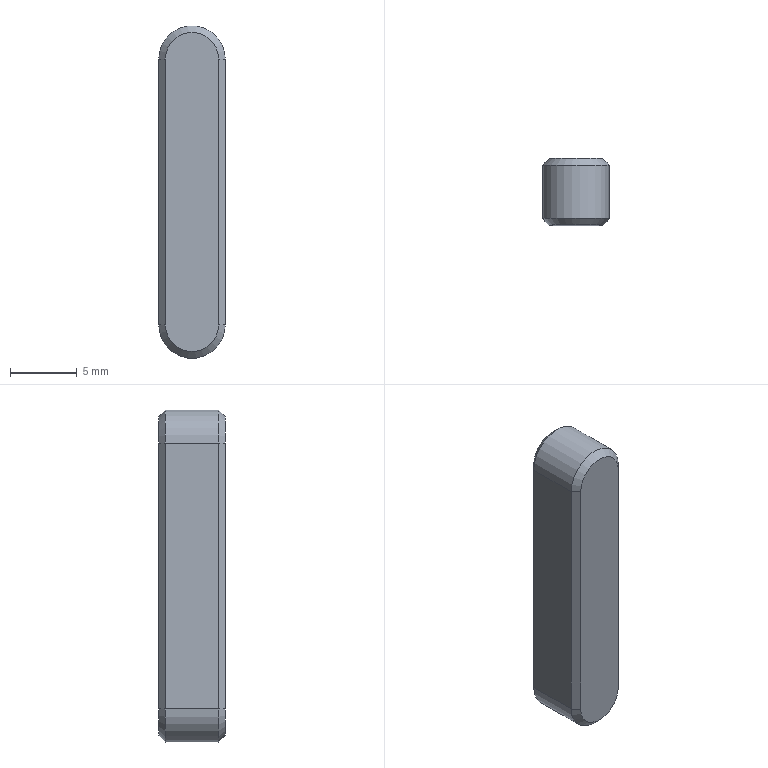Component | SolidWorks | 25x5x5ParallelKey-1 | 1 solid | 14 faces | box 5 x 5 x 25 mm | volume 585 mm3 | plane 8 | cone 4 | cylinder 2 | commonest cylinder face diameters 5 x2 | material AISI 1045 Steel, cold drawn
build123d program:
from build123d import *

# Parameters (mm, degrees)
BOSS_EXTRUDE1_DEPTH = 2.5
CHAMFER1_SIZE       = 0.5


with BuildPart() as part:
    # Sketch1 → Boss-Extrude1 (new, symmetric)
    with BuildSketch(Plane.XY):
        with BuildLine():
            Line((-2.5, -10), (-2.5, 10))
            ThreePointArc((-2.5, 10), (0, 12.5), (2.5, 10))
            Line((2.5, 10), (2.5, -10))
            ThreePointArc((2.5, -10), (0, -12.5), (-2.5, -10))
        make_face()
    extrude(amount=BOSS_EXTRUDE1_DEPTH, both=True)

    # Chamfer1
    chamfer1_edges = [part.edges().sort_by_distance(p)[0] for p in [
        (0, 12.5, 2.5),
        (-2.5, 0, 2.5),
        (0, -12.5, 2.5),
        (-2.5, 0, -2.5),
        (0, 12.5, -2.5),
        (2.5, 0, -2.5),
        (0, -12.5, -2.5),
        (2.5, 0, 2.5),
    ]]
    chamfer(chamfer1_edges, length=CHAMFER1_SIZE)


solid = part.part

# Placed as in the assembly
solid = solid.moved(Location((0, 7.5, 115.5), (90, 0, 0)))
STEP:
#1=CARTESIAN_POINT('',(-0.09843,0.2165,4.154));
#2=VERTEX_POINT('',#1);
#3=CARTESIAN_POINT('',(-0.09843,0.374,4.154));
#4=VERTEX_POINT('',#3);
#5=CARTESIAN_POINT('',(-0.09843,0.1969,4.154));
#6=DIRECTION('',(-0.,1.,-0.));
#7=VECTOR('',#6,39.37);
#8=LINE('',#5,#7);
#9=EDGE_CURVE('',#2,#4,#8,.T.);
#10=ORIENTED_EDGE('',*,*,#9,.T.);
#11=CARTESIAN_POINT('',(0.09843,0.374,4.154));
#12=VERTEX_POINT('',#11);
#13=CARTESIAN_POINT('',(-0.,0.374,4.154));
#14=DIRECTION('',(0.,-1.,0.));
#15=DIRECTION('',(1.,0.,0.));
#16=AXIS2_PLACEMENT_3D('',#13,#14,#15);
#17=CIRCLE('',#16,0.09843);
#18=EDGE_CURVE('',#4,#12,#17,.T.);
#19=ORIENTED_EDGE('',*,*,#18,.T.);
#20=CARTESIAN_POINT('',(0.09843,0.2165,4.154));
#21=VERTEX_POINT('',#20);
#22=CARTESIAN_POINT('',(0.09843,0.1969,4.154));
#23=DIRECTION('',(-0.,1.,-0.));
#24=VECTOR('',#23,39.37);
#25=LINE('',#22,#24);
#26=EDGE_CURVE('',#21,#12,#25,.T.);
#27=ORIENTED_EDGE('',*,*,#26,.F.);
#28=CARTESIAN_POINT('',(0.,0.2165,4.154));
#29=DIRECTION('',(-0.,1.,-0.));
#30=DIRECTION('',(1.,0.,0.));
#31=AXIS2_PLACEMENT_3D('',#28,#29,#30);
#32=CIRCLE('',#31,0.09843);
#33=EDGE_CURVE('',#21,#2,#32,.T.);
#34=ORIENTED_EDGE('',*,*,#33,.T.);
#35=EDGE_LOOP('',(#10,#19,#27,#34));
#36=FACE_OUTER_BOUND('',#35,.T.);
#37=CARTESIAN_POINT('',(0.,0.1969,4.154));
#38=DIRECTION('',(-0.,1.,-0.));
#39=DIRECTION('',(-1.,-0.,0.));
#40=AXIS2_PLACEMENT_3D('',#37,#38,#39);
#41=CYLINDRICAL_SURFACE('',#40,0.09843);
#42=ADVANCED_FACE('',(#36),#41,.T.);
#43=ORIENTED_EDGE('',*,*,#26,.T.);
#44=CARTESIAN_POINT('',(0.09843,0.374,4.941));
#45=VERTEX_POINT('',#44);
#46=CARTESIAN_POINT('',(0.09843,0.374,4.154));
#47=DIRECTION('',(0.,0.,1.));
#48=VECTOR('',#47,39.37);
#49=LINE('',#46,#48);
#50=EDGE_CURVE('',#12,#45,#49,.T.);
#51=ORIENTED_EDGE('',*,*,#50,.T.);
#52=CARTESIAN_POINT('',(0.09843,0.2165,4.941));
#53=VERTEX_POINT('',#52);
#54=CARTESIAN_POINT('',(0.09843,0.1969,4.941));
#55=DIRECTION('',(-0.,1.,-0.));
#56=VECTOR('',#55,39.37);
#57=LINE('',#54,#56);
#58=EDGE_CURVE('',#53,#45,#57,.T.);
#59=ORIENTED_EDGE('',*,*,#58,.F.);
#60=CARTESIAN_POINT('',(0.09843,0.2165,4.154));
#61=DIRECTION('',(-0.,-0.,-1.));
#62=VECTOR('',#61,39.37);
#63=LINE('',#60,#62);
#64=EDGE_CURVE('',#53,#21,#63,.T.);
#65=ORIENTED_EDGE('',*,*,#64,.T.);
#66=EDGE_LOOP('',(#43,#51,#59,#65));
#67=FACE_OUTER_BOUND('',#66,.T.);
#68=CARTESIAN_POINT('',(0.09843,0.1969,4.154));
#69=DIRECTION('',(-1.,-0.,0.));
#70=DIRECTION('',(-0.,-0.,-1.));
#71=AXIS2_PLACEMENT_3D('',#68,#69,#70);
#72=PLANE('',#71);
#73=ADVANCED_FACE('',(#67),#72,.F.);
#74=ORIENTED_EDGE('',*,*,#58,.T.);
#75=CARTESIAN_POINT('',(-0.09843,0.374,4.941));
#76=VERTEX_POINT('',#75);
#77=CARTESIAN_POINT('',(-0.,0.374,4.941));
#78=DIRECTION('',(0.,-1.,0.));
#79=DIRECTION('',(1.,0.,0.));
#80=AXIS2_PLACEMENT_3D('',#77,#78,#79);
#81=CIRCLE('',#80,0.09843);
#82=EDGE_CURVE('',#45,#76,#81,.T.);
#83=ORIENTED_EDGE('',*,*,#82,.T.);
#84=CARTESIAN_POINT('',(-0.09843,0.2165,4.941));
#85=VERTEX_POINT('',#84);
#86=CARTESIAN_POINT('',(-0.09843,0.1969,4.941));
#87=DIRECTION('',(-0.,1.,-0.));
#88=VECTOR('',#87,39.37);
#89=LINE('',#86,#88);
#90=EDGE_CURVE('',#85,#76,#89,.T.);
#91=ORIENTED_EDGE('',*,*,#90,.F.);
#92=CARTESIAN_POINT('',(0.,0.2165,4.941));
#93=DIRECTION('',(-0.,1.,-0.));
#94=DIRECTION('',(1.,0.,0.));
#95=AXIS2_PLACEMENT_3D('',#92,#93,#94);
#96=CIRCLE('',#95,0.09843);
#97=EDGE_CURVE('',#85,#53,#96,.T.);
#98=ORIENTED_EDGE('',*,*,#97,.T.);
#99=EDGE_LOOP('',(#74,#83,#91,#98));
#100=FACE_OUTER_BOUND('',#99,.T.);
#101=CARTESIAN_POINT('',(0.,0.1969,4.941));
#102=DIRECTION('',(-0.,1.,-0.));
#103=DIRECTION('',(-1.,-0.,0.));
#104=AXIS2_PLACEMENT_3D('',#101,#102,#103);
#105=CYLINDRICAL_SURFACE('',#104,0.09843);
#106=ADVANCED_FACE('',(#100),#105,.T.);
#107=ORIENTED_EDGE('',*,*,#90,.T.);
#108=CARTESIAN_POINT('',(-0.09843,0.374,4.154));
#109=DIRECTION('',(-0.,-0.,-1.));
#110=VECTOR('',#109,39.37);
#111=LINE('',#108,#110);
#112=EDGE_CURVE('',#76,#4,#111,.T.);
#113=ORIENTED_EDGE('',*,*,#112,.T.);
#114=ORIENTED_EDGE('',*,*,#9,.F.);
#115=CARTESIAN_POINT('',(-0.09843,0.2165,4.941));
#116=DIRECTION('',(0.,0.,1.));
#117=VECTOR('',#116,39.37);
#118=LINE('',#115,#117);
#119=EDGE_CURVE('',#2,#85,#118,.T.);
#120=ORIENTED_EDGE('',*,*,#119,.T.);
#121=EDGE_LOOP('',(#107,#113,#114,#120));
#122=FACE_OUTER_BOUND('',#121,.T.);
#123=CARTESIAN_POINT('',(-0.09843,0.1969,4.154));
#124=DIRECTION('',(1.,0.,-0.));
#125=DIRECTION('',(0.,0.,1.));
#126=AXIS2_PLACEMENT_3D('',#123,#124,#125);
#127=PLANE('',#126);
#128=ADVANCED_FACE('',(#122),#127,.F.);
#129=CARTESIAN_POINT('',(0.07874,0.1969,4.941));
#130=VERTEX_POINT('',#129);
#131=CARTESIAN_POINT('',(-0.07874,0.1969,4.941));
#132=VERTEX_POINT('',#131);
#133=CARTESIAN_POINT('',(0.,0.1969,4.941));
#134=DIRECTION('',(0.,-1.,0.));
#135=DIRECTION('',(1.,0.,0.));
#136=AXIS2_PLACEMENT_3D('',#133,#134,#135);
#137=CIRCLE('',#136,0.07874);
#138=EDGE_CURVE('',#130,#132,#137,.T.);
#139=ORIENTED_EDGE('',*,*,#138,.T.);
#140=CARTESIAN_POINT('',(-0.07874,0.1969,4.154));
#141=VERTEX_POINT('',#140);
#142=CARTESIAN_POINT('',(-0.07874,0.1969,4.154));
#143=DIRECTION('',(-0.,-0.,-1.));
#144=VECTOR('',#143,39.37);
#145=LINE('',#142,#144);
#146=EDGE_CURVE('',#132,#141,#145,.T.);
#147=ORIENTED_EDGE('',*,*,#146,.T.);
#148=CARTESIAN_POINT('',(0.07874,0.1969,4.154));
#149=VERTEX_POINT('',#148);
#150=CARTESIAN_POINT('',(0.,0.1969,4.154));
#151=DIRECTION('',(0.,-1.,0.));
#152=DIRECTION('',(1.,0.,0.));
#153=AXIS2_PLACEMENT_3D('',#150,#151,#152);
#154=CIRCLE('',#153,0.07874);
#155=EDGE_CURVE('',#141,#149,#154,.T.);
#156=ORIENTED_EDGE('',*,*,#155,.T.);
#157=CARTESIAN_POINT('',(0.07874,0.1969,4.941));
#158=DIRECTION('',(0.,0.,1.));
#159=VECTOR('',#158,39.37);
#160=LINE('',#157,#159);
#161=EDGE_CURVE('',#149,#130,#160,.T.);
#162=ORIENTED_EDGE('',*,*,#161,.T.);
#163=EDGE_LOOP('',(#139,#147,#156,#162));
#164=FACE_OUTER_BOUND('',#163,.T.);
#165=CARTESIAN_POINT('',(0.,0.1969,4.154));
#166=DIRECTION('',(0.,-1.,0.));
#167=DIRECTION('',(1.,0.,-0.));
#168=AXIS2_PLACEMENT_3D('',#165,#166,#167);
#169=PLANE('',#168);
#170=ADVANCED_FACE('',(#164),#169,.T.);
#171=CARTESIAN_POINT('',(-0.07874,0.3937,4.941));
#172=VERTEX_POINT('',#171);
#173=CARTESIAN_POINT('',(0.07874,0.3937,4.941));
#174=VERTEX_POINT('',#173);
#175=CARTESIAN_POINT('',(-0.,0.3937,4.941));
#176=DIRECTION('',(-0.,1.,-0.));
#177=DIRECTION('',(1.,0.,0.));
#178=AXIS2_PLACEMENT_3D('',#175,#176,#177);
#179=CIRCLE('',#178,0.07874);
#180=EDGE_CURVE('',#172,#174,#179,.T.);
#181=ORIENTED_EDGE('',*,*,#180,.T.);
#182=CARTESIAN_POINT('',(0.07874,0.3937,4.154));
#183=VERTEX_POINT('',#182);
#184=CARTESIAN_POINT('',(0.07874,0.3937,4.154));
#185=DIRECTION('',(-0.,-0.,-1.));
#186=VECTOR('',#185,39.37);
#187=LINE('',#184,#186);
#188=EDGE_CURVE('',#174,#183,#187,.T.);
#189=ORIENTED_EDGE('',*,*,#188,.T.);
#190=CARTESIAN_POINT('',(-0.07874,0.3937,4.154));
#191=VERTEX_POINT('',#190);
#192=CARTESIAN_POINT('',(-0.,0.3937,4.154));
#193=DIRECTION('',(-0.,1.,-0.));
#194=DIRECTION('',(1.,0.,0.));
#195=AXIS2_PLACEMENT_3D('',#192,#193,#194);
#196=CIRCLE('',#195,0.07874);
#197=EDGE_CURVE('',#183,#191,#196,.T.);
#198=ORIENTED_EDGE('',*,*,#197,.T.);
#199=CARTESIAN_POINT('',(-0.07874,0.3937,4.154));
#200=DIRECTION('',(0.,0.,1.));
#201=VECTOR('',#200,39.37);
#202=LINE('',#199,#201);
#203=EDGE_CURVE('',#191,#172,#202,.T.);
#204=ORIENTED_EDGE('',*,*,#203,.T.);
#205=EDGE_LOOP('',(#181,#189,#198,#204));
#206=FACE_OUTER_BOUND('',#205,.T.);
#207=CARTESIAN_POINT('',(-0.,0.3937,4.154));
#208=DIRECTION('',(0.,-1.,0.));
#209=DIRECTION('',(1.,0.,-0.));
#210=AXIS2_PLACEMENT_3D('',#207,#208,#209);
#211=PLANE('',#210);
#212=ADVANCED_FACE('',(#206),#211,.F.);
#213=CARTESIAN_POINT('',(-0.07874,0.3937,4.941));
#214=DIRECTION('',(-0.7071,-0.7071,0.));
#215=VECTOR('',#214,39.37);
#216=LINE('',#213,#215);
#217=EDGE_CURVE('',#172,#76,#216,.T.);
#218=ORIENTED_EDGE('',*,*,#217,.F.);
#219=ORIENTED_EDGE('',*,*,#203,.F.);
#220=CARTESIAN_POINT('',(-0.09843,0.374,4.154));
#221=DIRECTION('',(0.7071,0.7071,-0.));
#222=VECTOR('',#221,39.37);
#223=LINE('',#220,#222);
#224=EDGE_CURVE('',#4,#191,#223,.T.);
#225=ORIENTED_EDGE('',*,*,#224,.F.);
#226=ORIENTED_EDGE('',*,*,#112,.F.);
#227=EDGE_LOOP('',(#218,#219,#225,#226));
#228=FACE_OUTER_BOUND('',#227,.T.);
#229=CARTESIAN_POINT('',(-0.09843,0.374,4.154));
#230=DIRECTION('',(0.7071,-0.7071,-0.));
#231=DIRECTION('',(-0.,-0.,-1.));
#232=AXIS2_PLACEMENT_3D('',#229,#230,#231);
#233=PLANE('',#232);
#234=ADVANCED_FACE('',(#228),#233,.F.);
#235=ORIENTED_EDGE('',*,*,#224,.T.);
#236=ORIENTED_EDGE('',*,*,#197,.F.);
#237=CARTESIAN_POINT('',(0.09843,0.374,4.154));
#238=DIRECTION('',(-0.7071,0.7071,0.));
#239=VECTOR('',#238,39.37);
#240=LINE('',#237,#239);
#241=EDGE_CURVE('',#12,#183,#240,.T.);
#242=ORIENTED_EDGE('',*,*,#241,.F.);
#243=ORIENTED_EDGE('',*,*,#18,.F.);
#244=EDGE_LOOP('',(#235,#236,#242,#243));
#245=FACE_OUTER_BOUND('',#244,.T.);
#246=CARTESIAN_POINT('',(-0.,0.374,4.154));
#247=DIRECTION('',(0.,-1.,0.));
#248=DIRECTION('',(1.,0.,0.));
#249=AXIS2_PLACEMENT_3D('',#246,#247,#248);
#250=CONICAL_SURFACE('',#249,0.09843,0.7854);
#251=ADVANCED_FACE('',(#245),#250,.T.);
#252=ORIENTED_EDGE('',*,*,#217,.T.);
#253=ORIENTED_EDGE('',*,*,#82,.F.);
#254=CARTESIAN_POINT('',(0.07874,0.3937,4.941));
#255=DIRECTION('',(0.7071,-0.7071,-0.));
#256=VECTOR('',#255,39.37);
#257=LINE('',#254,#256);
#258=EDGE_CURVE('',#174,#45,#257,.T.);
#259=ORIENTED_EDGE('',*,*,#258,.F.);
#260=ORIENTED_EDGE('',*,*,#180,.F.);
#261=EDGE_LOOP('',(#252,#253,#259,#260));
#262=FACE_OUTER_BOUND('',#261,.T.);
#263=CARTESIAN_POINT('',(-0.,0.374,4.941));
#264=DIRECTION('',(0.,-1.,0.));
#265=DIRECTION('',(1.,0.,0.));
#266=AXIS2_PLACEMENT_3D('',#263,#264,#265);
#267=CONICAL_SURFACE('',#266,0.09843,0.7854);
#268=ADVANCED_FACE('',(#262),#267,.T.);
#269=ORIENTED_EDGE('',*,*,#241,.T.);
#270=ORIENTED_EDGE('',*,*,#188,.F.);
#271=ORIENTED_EDGE('',*,*,#258,.T.);
#272=ORIENTED_EDGE('',*,*,#50,.F.);
#273=EDGE_LOOP('',(#269,#270,#271,#272));
#274=FACE_OUTER_BOUND('',#273,.T.);
#275=CARTESIAN_POINT('',(0.09843,0.374,4.154));
#276=DIRECTION('',(-0.7071,-0.7071,0.));
#277=DIRECTION('',(0.,0.,1.));
#278=AXIS2_PLACEMENT_3D('',#275,#276,#277);
#279=PLANE('',#278);
#280=ADVANCED_FACE('',(#274),#279,.F.);
#281=CARTESIAN_POINT('',(0.09843,0.2165,4.154));
#282=DIRECTION('',(-0.7071,-0.7071,0.));
#283=VECTOR('',#282,39.37);
#284=LINE('',#281,#283);
#285=EDGE_CURVE('',#21,#149,#284,.T.);
#286=ORIENTED_EDGE('',*,*,#285,.F.);
#287=ORIENTED_EDGE('',*,*,#64,.F.);
#288=CARTESIAN_POINT('',(0.07874,0.1969,4.941));
#289=DIRECTION('',(0.7071,0.7071,-0.));
#290=VECTOR('',#289,39.37);
#291=LINE('',#288,#290);
#292=EDGE_CURVE('',#130,#53,#291,.T.);
#293=ORIENTED_EDGE('',*,*,#292,.F.);
#294=ORIENTED_EDGE('',*,*,#161,.F.);
#295=EDGE_LOOP('',(#286,#287,#293,#294));
#296=FACE_OUTER_BOUND('',#295,.T.);
#297=CARTESIAN_POINT('',(0.07874,0.1969,4.154));
#298=DIRECTION('',(0.7071,-0.7071,-0.));
#299=DIRECTION('',(-0.,-0.,-1.));
#300=AXIS2_PLACEMENT_3D('',#297,#298,#299);
#301=PLANE('',#300);
#302=ADVANCED_FACE('',(#296),#301,.T.);
#303=ORIENTED_EDGE('',*,*,#292,.T.);
#304=ORIENTED_EDGE('',*,*,#97,.F.);
#305=CARTESIAN_POINT('',(-0.07874,0.1969,4.941));
#306=DIRECTION('',(-0.7071,0.7071,0.));
#307=VECTOR('',#306,39.37);
#308=LINE('',#305,#307);
#309=EDGE_CURVE('',#132,#85,#308,.T.);
#310=ORIENTED_EDGE('',*,*,#309,.F.);
#311=ORIENTED_EDGE('',*,*,#138,.F.);
#312=EDGE_LOOP('',(#303,#304,#310,#311));
#313=FACE_OUTER_BOUND('',#312,.T.);
#314=CARTESIAN_POINT('',(0.,0.1969,4.941));
#315=DIRECTION('',(-0.,1.,-0.));
#316=DIRECTION('',(-1.,-0.,0.));
#317=AXIS2_PLACEMENT_3D('',#314,#315,#316);
#318=CONICAL_SURFACE('',#317,0.07874,0.7854);
#319=ADVANCED_FACE('',(#313),#318,.T.);
#320=ORIENTED_EDGE('',*,*,#285,.T.);
#321=ORIENTED_EDGE('',*,*,#155,.F.);
#322=CARTESIAN_POINT('',(-0.09843,0.2165,4.154));
#323=DIRECTION('',(0.7071,-0.7071,-0.));
#324=VECTOR('',#323,39.37);
#325=LINE('',#322,#324);
#326=EDGE_CURVE('',#2,#141,#325,.T.);
#327=ORIENTED_EDGE('',*,*,#326,.F.);
#328=ORIENTED_EDGE('',*,*,#33,.F.);
#329=EDGE_LOOP('',(#320,#321,#327,#328));
#330=FACE_OUTER_BOUND('',#329,.T.);
#331=CARTESIAN_POINT('',(0.,0.1969,4.154));
#332=DIRECTION('',(-0.,1.,-0.));
#333=DIRECTION('',(-1.,-0.,0.));
#334=AXIS2_PLACEMENT_3D('',#331,#332,#333);
#335=CONICAL_SURFACE('',#334,0.07874,0.7854);
#336=ADVANCED_FACE('',(#330),#335,.T.);
#337=ORIENTED_EDGE('',*,*,#309,.T.);
#338=ORIENTED_EDGE('',*,*,#119,.F.);
#339=ORIENTED_EDGE('',*,*,#326,.T.);
#340=ORIENTED_EDGE('',*,*,#146,.F.);
#341=EDGE_LOOP('',(#337,#338,#339,#340));
#342=FACE_OUTER_BOUND('',#341,.T.);
#343=CARTESIAN_POINT('',(-0.07874,0.1969,4.154));
#344=DIRECTION('',(-0.7071,-0.7071,0.));
#345=DIRECTION('',(0.,0.,1.));
#346=AXIS2_PLACEMENT_3D('',#343,#344,#345);
#347=PLANE('',#346);
#348=ADVANCED_FACE('',(#342),#347,.T.);
#349=CLOSED_SHELL('',(#42,#73,#106,#128,#170,#212,#234,#251,#268,#280,#302,#319,#336,#348));
#350=MANIFOLD_SOLID_BREP('',#349);
#351=CARTESIAN_POINT('',(0.,0.,0.));
#352=DIRECTION('',(0.,0.,1.));
#353=DIRECTION('',(1.,0.,0.));
#354=AXIS2_PLACEMENT_3D('',#351,#352,#353);
#355=(LENGTH_UNIT()NAMED_UNIT(*)SI_UNIT($,.METRE.));
#356=LENGTH_MEASURE_WITH_UNIT(LENGTH_MEASURE(0.0254),#355);
#357=DIMENSIONAL_EXPONENTS(1.,0.,0.,0.,0.,0.,0.);
#358=(CONVERSION_BASED_UNIT('',#356)LENGTH_UNIT()NAMED_UNIT(#357));
#359=UNCERTAINTY_MEASURE_WITH_UNIT(LENGTH_MEASURE(0.00001),#358,'','');
#360=(NAMED_UNIT(*)PLANE_ANGLE_UNIT()SI_UNIT($,.RADIAN.));
#361=(NAMED_UNIT(*)SI_UNIT($,.STERADIAN.)SOLID_ANGLE_UNIT());
#362=(GEOMETRIC_REPRESENTATION_CONTEXT(3)GLOBAL_UNCERTAINTY_ASSIGNED_CONTEXT((#359))GLOBAL_UNIT_ASSIGNED_CONTEXT((#358,#360,#361))REPRESENTATION_CONTEXT('',''));
#363=ADVANCED_BREP_SHAPE_REPRESENTATION('',(#350,#354),#362);
#364=COLOUR_RGB('',0.7922,0.8196,0.9333);
#365=FILL_AREA_STYLE_COLOUR('',#364);
#366=FILL_AREA_STYLE('',(#365));
#367=SURFACE_STYLE_FILL_AREA(#366);
#368=SURFACE_SIDE_STYLE('',(#367));
#369=SURFACE_STYLE_USAGE(.BOTH.,#368);
#370=PRESENTATION_STYLE_ASSIGNMENT((#369));
#371=STYLED_ITEM('',(#370),#350);
#372=(LENGTH_UNIT()NAMED_UNIT(*)SI_UNIT($,.METRE.));
#373=LENGTH_MEASURE_WITH_UNIT(LENGTH_MEASURE(0.0254),#372);
#374=DIMENSIONAL_EXPONENTS(1.,0.,0.,0.,0.,0.,0.);
#375=(CONVERSION_BASED_UNIT('',#373)LENGTH_UNIT()NAMED_UNIT(#374));
#376=UNCERTAINTY_MEASURE_WITH_UNIT(LENGTH_MEASURE(0.00001),#375,'','');
#377=(NAMED_UNIT(*)PLANE_ANGLE_UNIT()SI_UNIT($,.RADIAN.));
#378=(NAMED_UNIT(*)SI_UNIT($,.STERADIAN.)SOLID_ANGLE_UNIT());
#379=(GEOMETRIC_REPRESENTATION_CONTEXT(3)GLOBAL_UNCERTAINTY_ASSIGNED_CONTEXT((#376))GLOBAL_UNIT_ASSIGNED_CONTEXT((#375,#377,#378))REPRESENTATION_CONTEXT('',''));
#380=MECHANICAL_DESIGN_GEOMETRIC_PRESENTATION_REPRESENTATION('',(#371),#379);
#381=PRESENTATION_LAYER_ASSIGNMENT('','',(#371));